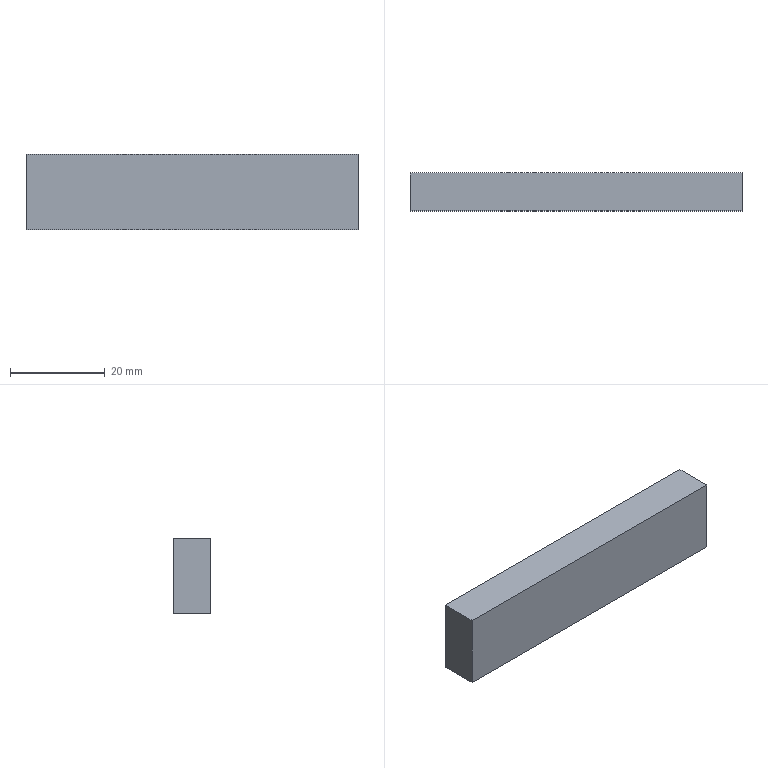Component | SolidWorks | SiliconeShockAbsorberBlock-1 | 1 solid | 6 faces | box 70 x 8 x 16 mm | volume 8960 mm3 | plane 6
build123d program:
from build123d import *

# Parameters (mm, degrees)
SKETCH1_W           = 70
SKETCH1_H           = 8
BOSS_EXTRUDE1_DEPTH = 8


with BuildPart() as part:
    # Sketch1 → Boss-Extrude1 (new, symmetric)
    with BuildSketch(Plane.XY):
        with Locations((35, 4)):
            Rectangle(SKETCH1_W, SKETCH1_H)
    extrude(amount=BOSS_EXTRUDE1_DEPTH, both=True)


solid = part.part

# Placed as in the assembly
solid = solid.moved(Location((29.354, -42.068, 156.933), (0, 0, 0)))
STEP:
#1=COLOUR_RGB('',0.7922,0.8196,0.9333);
#2=FILL_AREA_STYLE_COLOUR('',#1);
#3=FILL_AREA_STYLE('',(#2));
#4=SURFACE_STYLE_FILL_AREA(#3);
#5=SURFACE_SIDE_STYLE('',(#4));
#6=SURFACE_STYLE_USAGE(.BOTH.,#5);
#7=PRESENTATION_STYLE_ASSIGNMENT((#6));
#8=CARTESIAN_POINT('',(1.156,-1.341,5.863));
#9=VERTEX_POINT('',#8);
#10=CARTESIAN_POINT('',(1.156,-1.656,5.863));
#11=VERTEX_POINT('',#10);
#12=CARTESIAN_POINT('',(1.156,-1.656,5.863));
#13=DIRECTION('',(0.,-1.,0.));
#14=VECTOR('',#13,39.37);
#15=LINE('',#12,#14);
#16=EDGE_CURVE('',#9,#11,#15,.T.);
#17=ORIENTED_EDGE('',*,*,#16,.T.);
#18=CARTESIAN_POINT('',(1.156,-1.656,6.493));
#19=VERTEX_POINT('',#18);
#20=CARTESIAN_POINT('',(1.156,-1.656,6.493));
#21=DIRECTION('',(0.,0.,-1.));
#22=VECTOR('',#21,39.37);
#23=LINE('',#20,#22);
#24=EDGE_CURVE('',#19,#11,#23,.T.);
#25=ORIENTED_EDGE('',*,*,#24,.F.);
#26=CARTESIAN_POINT('',(1.156,-1.341,6.493));
#27=VERTEX_POINT('',#26);
#28=CARTESIAN_POINT('',(1.156,-1.656,6.493));
#29=DIRECTION('',(0.,-1.,0.));
#30=VECTOR('',#29,39.37);
#31=LINE('',#28,#30);
#32=EDGE_CURVE('',#27,#19,#31,.T.);
#33=ORIENTED_EDGE('',*,*,#32,.F.);
#34=CARTESIAN_POINT('',(1.156,-1.341,6.493));
#35=DIRECTION('',(0.,0.,-1.));
#36=VECTOR('',#35,39.37);
#37=LINE('',#34,#36);
#38=EDGE_CURVE('',#27,#9,#37,.T.);
#39=ORIENTED_EDGE('',*,*,#38,.T.);
#40=EDGE_LOOP('',(#17,#25,#33,#39));
#41=FACE_OUTER_BOUND('',#40,.T.);
#42=CARTESIAN_POINT('',(1.156,-1.656,6.493));
#43=DIRECTION('',(1.,0.,0.));
#44=DIRECTION('',(0.,0.,-1.));
#45=AXIS2_PLACEMENT_3D('',#42,#43,#44);
#46=PLANE('',#45);
#47=ADVANCED_FACE('',(#41),#46,.F.);
#48=CARTESIAN_POINT('',(3.912,-1.656,5.863));
#49=VERTEX_POINT('',#48);
#50=CARTESIAN_POINT('',(1.156,-1.656,5.863));
#51=DIRECTION('',(1.,0.,0.));
#52=VECTOR('',#51,39.37);
#53=LINE('',#50,#52);
#54=EDGE_CURVE('',#11,#49,#53,.T.);
#55=ORIENTED_EDGE('',*,*,#54,.T.);
#56=CARTESIAN_POINT('',(3.912,-1.656,6.493));
#57=VERTEX_POINT('',#56);
#58=CARTESIAN_POINT('',(3.912,-1.656,6.493));
#59=DIRECTION('',(0.,0.,-1.));
#60=VECTOR('',#59,39.37);
#61=LINE('',#58,#60);
#62=EDGE_CURVE('',#57,#49,#61,.T.);
#63=ORIENTED_EDGE('',*,*,#62,.F.);
#64=CARTESIAN_POINT('',(1.156,-1.656,6.493));
#65=DIRECTION('',(1.,0.,0.));
#66=VECTOR('',#65,39.37);
#67=LINE('',#64,#66);
#68=EDGE_CURVE('',#19,#57,#67,.T.);
#69=ORIENTED_EDGE('',*,*,#68,.F.);
#70=ORIENTED_EDGE('',*,*,#24,.T.);
#71=EDGE_LOOP('',(#55,#63,#69,#70));
#72=FACE_OUTER_BOUND('',#71,.T.);
#73=CARTESIAN_POINT('',(1.156,-1.656,6.493));
#74=DIRECTION('',(0.,1.,0.));
#75=DIRECTION('',(0.,0.,1.));
#76=AXIS2_PLACEMENT_3D('',#73,#74,#75);
#77=PLANE('',#76);
#78=ADVANCED_FACE('',(#72),#77,.F.);
#79=CARTESIAN_POINT('',(3.912,-1.341,5.863));
#80=VERTEX_POINT('',#79);
#81=CARTESIAN_POINT('',(3.912,-1.656,5.863));
#82=DIRECTION('',(0.,1.,0.));
#83=VECTOR('',#82,39.37);
#84=LINE('',#81,#83);
#85=EDGE_CURVE('',#49,#80,#84,.T.);
#86=ORIENTED_EDGE('',*,*,#85,.T.);
#87=CARTESIAN_POINT('',(3.912,-1.341,6.493));
#88=VERTEX_POINT('',#87);
#89=CARTESIAN_POINT('',(3.912,-1.341,6.493));
#90=DIRECTION('',(0.,0.,-1.));
#91=VECTOR('',#90,39.37);
#92=LINE('',#89,#91);
#93=EDGE_CURVE('',#88,#80,#92,.T.);
#94=ORIENTED_EDGE('',*,*,#93,.F.);
#95=CARTESIAN_POINT('',(3.912,-1.656,6.493));
#96=DIRECTION('',(0.,1.,0.));
#97=VECTOR('',#96,39.37);
#98=LINE('',#95,#97);
#99=EDGE_CURVE('',#57,#88,#98,.T.);
#100=ORIENTED_EDGE('',*,*,#99,.F.);
#101=ORIENTED_EDGE('',*,*,#62,.T.);
#102=EDGE_LOOP('',(#86,#94,#100,#101));
#103=FACE_OUTER_BOUND('',#102,.T.);
#104=CARTESIAN_POINT('',(3.912,-1.656,6.493));
#105=DIRECTION('',(-1.,0.,0.));
#106=DIRECTION('',(0.,0.,1.));
#107=AXIS2_PLACEMENT_3D('',#104,#105,#106);
#108=PLANE('',#107);
#109=ADVANCED_FACE('',(#103),#108,.F.);
#110=CARTESIAN_POINT('',(1.156,-1.341,5.863));
#111=DIRECTION('',(-1.,0.,0.));
#112=VECTOR('',#111,39.37);
#113=LINE('',#110,#112);
#114=EDGE_CURVE('',#80,#9,#113,.T.);
#115=ORIENTED_EDGE('',*,*,#114,.T.);
#116=ORIENTED_EDGE('',*,*,#38,.F.);
#117=CARTESIAN_POINT('',(1.156,-1.341,6.493));
#118=DIRECTION('',(-1.,0.,0.));
#119=VECTOR('',#118,39.37);
#120=LINE('',#117,#119);
#121=EDGE_CURVE('',#88,#27,#120,.T.);
#122=ORIENTED_EDGE('',*,*,#121,.F.);
#123=ORIENTED_EDGE('',*,*,#93,.T.);
#124=EDGE_LOOP('',(#115,#116,#122,#123));
#125=FACE_OUTER_BOUND('',#124,.T.);
#126=CARTESIAN_POINT('',(1.156,-1.341,6.493));
#127=DIRECTION('',(0.,-1.,0.));
#128=DIRECTION('',(0.,0.,-1.));
#129=AXIS2_PLACEMENT_3D('',#126,#127,#128);
#130=PLANE('',#129);
#131=ADVANCED_FACE('',(#125),#130,.F.);
#132=ORIENTED_EDGE('',*,*,#32,.T.);
#133=ORIENTED_EDGE('',*,*,#68,.T.);
#134=ORIENTED_EDGE('',*,*,#99,.T.);
#135=ORIENTED_EDGE('',*,*,#121,.T.);
#136=EDGE_LOOP('',(#132,#133,#134,#135));
#137=FACE_OUTER_BOUND('',#136,.T.);
#138=CARTESIAN_POINT('',(1.156,-1.656,6.493));
#139=DIRECTION('',(0.,0.,-1.));
#140=DIRECTION('',(-1.,0.,0.));
#141=AXIS2_PLACEMENT_3D('',#138,#139,#140);
#142=PLANE('',#141);
#143=ADVANCED_FACE('',(#137),#142,.F.);
#144=ORIENTED_EDGE('',*,*,#16,.F.);
#145=ORIENTED_EDGE('',*,*,#114,.F.);
#146=ORIENTED_EDGE('',*,*,#85,.F.);
#147=ORIENTED_EDGE('',*,*,#54,.F.);
#148=EDGE_LOOP('',(#144,#145,#146,#147));
#149=FACE_OUTER_BOUND('',#148,.T.);
#150=CARTESIAN_POINT('',(1.156,-1.656,5.863));
#151=DIRECTION('',(0.,0.,-1.));
#152=DIRECTION('',(-1.,0.,0.));
#153=AXIS2_PLACEMENT_3D('',#150,#151,#152);
#154=PLANE('',#153);
#155=ADVANCED_FACE('',(#149),#154,.T.);
#156=CLOSED_SHELL('',(#47,#78,#109,#131,#143,#155));
#157=MANIFOLD_SOLID_BREP('',#156);
#158=STYLED_ITEM('',(#7),#157);
#159=(LENGTH_UNIT()NAMED_UNIT(*)SI_UNIT($,.METRE.));
#160=LENGTH_MEASURE_WITH_UNIT(LENGTH_MEASURE(0.0254),#159);
#161=DIMENSIONAL_EXPONENTS(1.,0.,0.,0.,0.,0.,0.);
#162=(CONVERSION_BASED_UNIT('',#160)LENGTH_UNIT()NAMED_UNIT(#161));
#163=UNCERTAINTY_MEASURE_WITH_UNIT(LENGTH_MEASURE(0.00001),#162,'','');
#164=(NAMED_UNIT(*)PLANE_ANGLE_UNIT()SI_UNIT($,.RADIAN.));
#165=(NAMED_UNIT(*)SI_UNIT($,.STERADIAN.)SOLID_ANGLE_UNIT());
#166=(GEOMETRIC_REPRESENTATION_CONTEXT(3)GLOBAL_UNCERTAINTY_ASSIGNED_CONTEXT((#163))GLOBAL_UNIT_ASSIGNED_CONTEXT((#162,#164,#165))REPRESENTATION_CONTEXT('',''));
#167=MECHANICAL_DESIGN_GEOMETRIC_PRESENTATION_REPRESENTATION('',(#158),#166);
#168=CARTESIAN_POINT('',(0.,0.,0.));
#169=DIRECTION('',(0.,0.,1.));
#170=DIRECTION('',(1.,0.,0.));
#171=AXIS2_PLACEMENT_3D('',#168,#169,#170);
#172=(LENGTH_UNIT()NAMED_UNIT(*)SI_UNIT($,.METRE.));
#173=LENGTH_MEASURE_WITH_UNIT(LENGTH_MEASURE(0.0254),#172);
#174=DIMENSIONAL_EXPONENTS(1.,0.,0.,0.,0.,0.,0.);
#175=(CONVERSION_BASED_UNIT('',#173)LENGTH_UNIT()NAMED_UNIT(#174));
#176=UNCERTAINTY_MEASURE_WITH_UNIT(LENGTH_MEASURE(0.00001),#175,'','');
#177=(NAMED_UNIT(*)PLANE_ANGLE_UNIT()SI_UNIT($,.RADIAN.));
#178=(NAMED_UNIT(*)SI_UNIT($,.STERADIAN.)SOLID_ANGLE_UNIT());
#179=(GEOMETRIC_REPRESENTATION_CONTEXT(3)GLOBAL_UNCERTAINTY_ASSIGNED_CONTEXT((#176))GLOBAL_UNIT_ASSIGNED_CONTEXT((#175,#177,#178))REPRESENTATION_CONTEXT('',''));
#180=ADVANCED_BREP_SHAPE_REPRESENTATION('',(#157,#171),#179);
#181=PRESENTATION_LAYER_ASSIGNMENT('','',(#158));